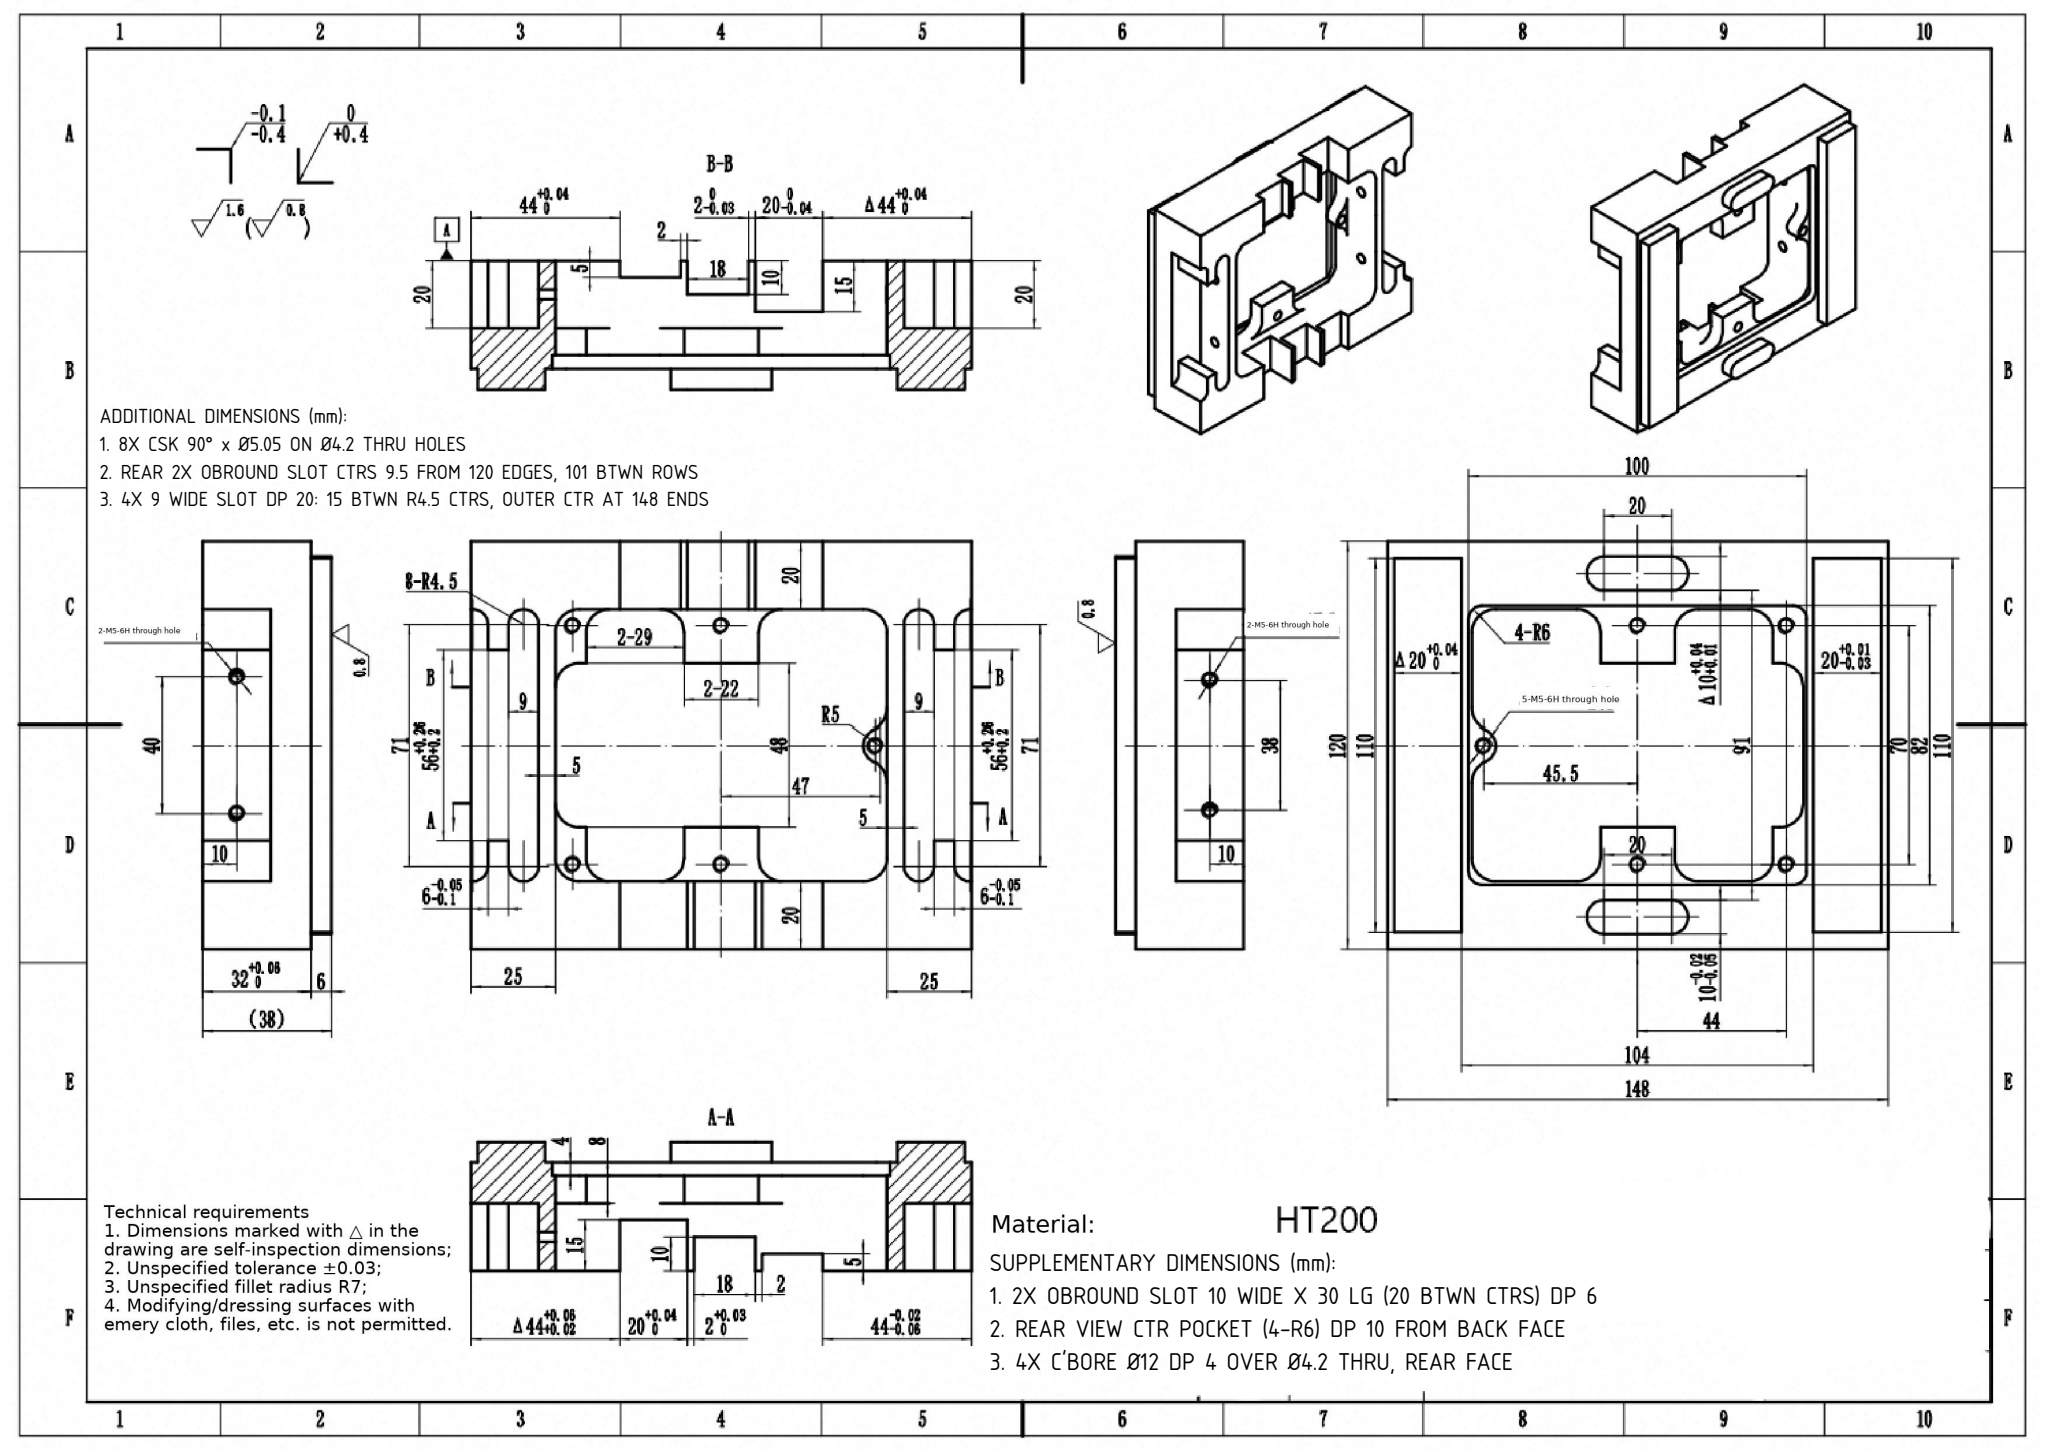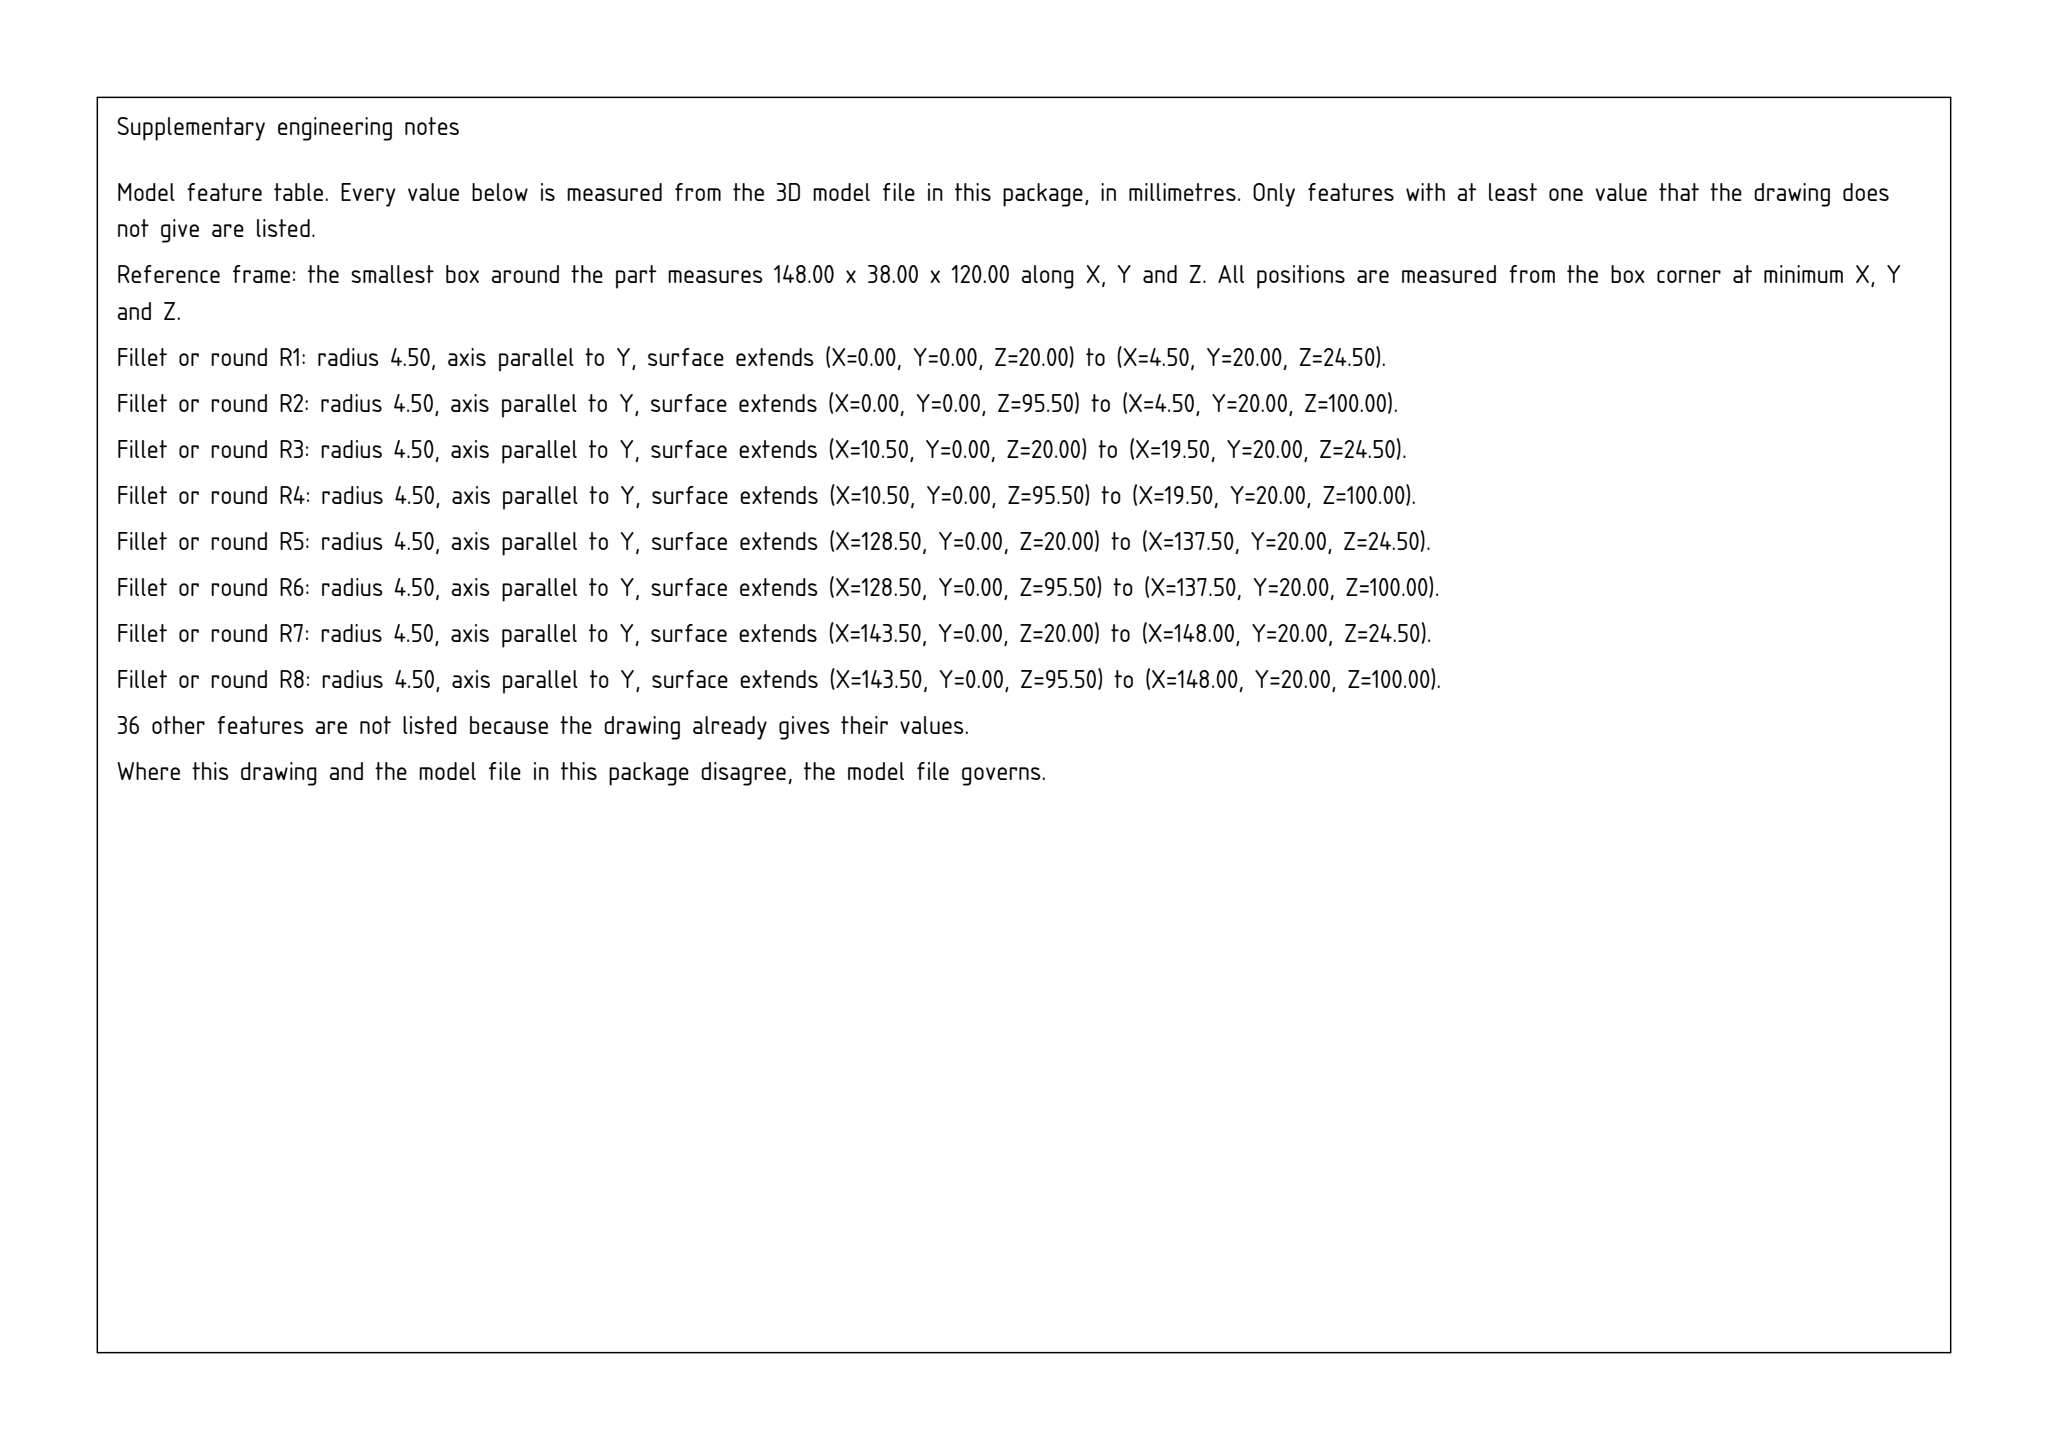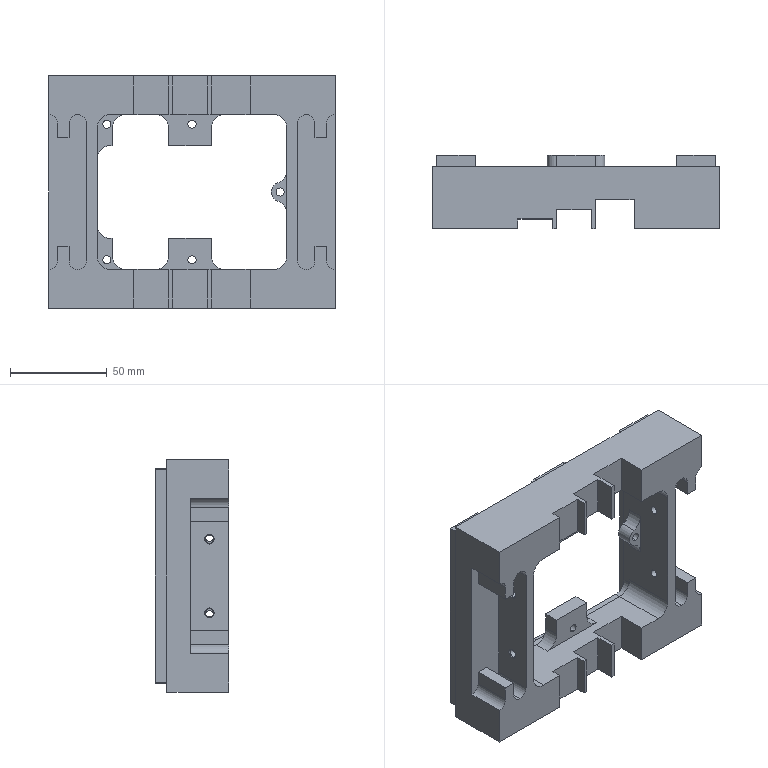Part | SolidWorks | mm | 1 solid | 144 faces | box 148 x 38 x 120 mm | volume 276636 mm3 | plane 85 | cylinder 51 | cone 8 | commonest cylinder face diameters 4.2 x18 14 x14 9 x10 10 x5 12 x4